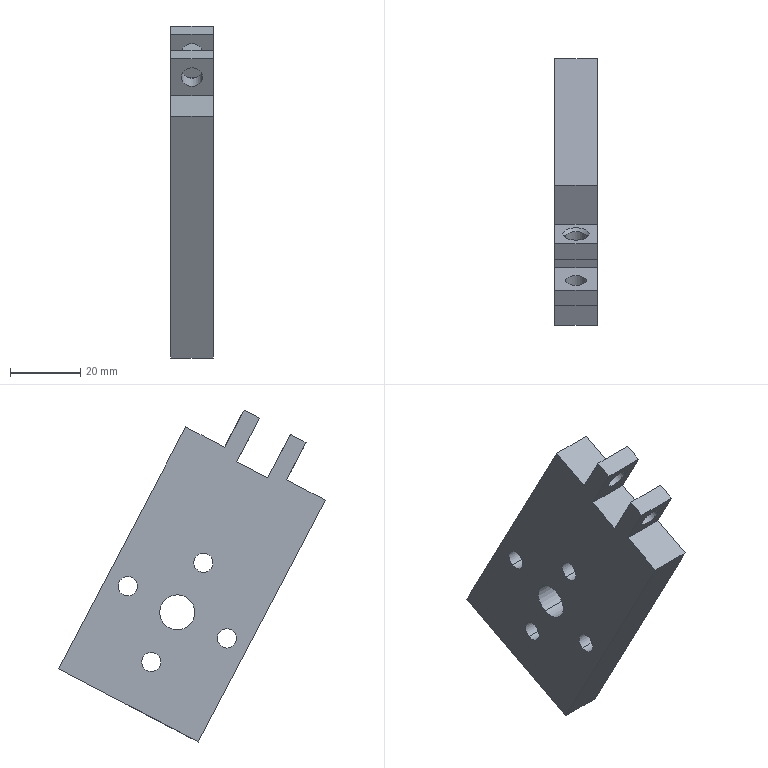Component | SolidWorks | RotaryCylinderFixingPlate-1 | 1 solid | 50 faces | box 12 x 76.1 x 94.79 mm | volume 39022 mm3 | cylinder 26 | plane 18 | cone 6 | commonest cylinder face diameters 10 x10 5.5 x8 4.2 x4 6 x4
build123d program:
from build123d import *

# Parameters (mm, degrees)
SKETCH1_W                                          = 90
SKETCH1_H                                          = 45
BOSS_EXTRUDE1_DEPTH                                = 12
HOLE_SIZE_ACCORDING_TO_TYPE_1_OF_HEXAG_D           = 5.5
HOLE_SIZE_ACCORDING_TO_TYPE_1_OF_HEXAG_CBORE_D     = 10
HOLE_SIZE_ACCORDING_TO_TYPE_1_OF_HEXAG_CBORE_DEPTH = 5.7
SKETCH5_R                                          = 5
CUT_EXTRUDE1_DEPTH                                 = 52.723
SKETCH6_W                                          = 12
SKETCH6_H                                          = 12.5
CUT_EXTRUDE2_DEPTH                                 = 52.723
SKETCH7_W                                          = 28
SKETCH7_H                                          = 10
CUT_EXTRUDE3_DEPTH                                 = 52.723
F_6_0_6_DIAMETER_HOLE1_D                           = 6
M5_TAPPED_HOLE1_D                                  = 4.2
M5_TAPPED_HOLE1_DEPTH                              = 24
M5_TAPPED_HOLE1_TIP                                = 1.262
CHAMFER1_SIZE                                      = 0.8


with BuildPart() as part:
    # Sketch1 → Boss-Extrude1 (new body)
    with BuildSketch(Plane.XY):
        Rectangle(SKETCH1_W, SKETCH1_H)
    extrude(amount=BOSS_EXTRUDE1_DEPTH)

    # Hole Size _according to_ Type 1 of Hexag (through all)
    with Locations(Plane.XY.offset(12)):
        with Locations((15, 16), (15, -16), (31, 0), (-1, 0)):
            CounterBoreHole(HOLE_SIZE_ACCORDING_TO_TYPE_1_OF_HEXAG_D / 2, HOLE_SIZE_ACCORDING_TO_TYPE_1_OF_HEXAG_CBORE_D / 2, HOLE_SIZE_ACCORDING_TO_TYPE_1_OF_HEXAG_CBORE_DEPTH)

    # Sketch5 → Cut-Extrude1 (cut, through all)
    with BuildSketch(Plane.XY.offset(12)):
        with Locations((15, 0)):
            Circle(SKETCH5_R)
    extrude(amount=-CUT_EXTRUDE1_DEPTH, mode=Mode.SUBTRACT)

    # Sketch6 → Cut-Extrude2 (cut, through all)
    with BuildSketch(Plane.XY.offset(12)):
        with Locations((-39, 16.25)):
            Rectangle(SKETCH6_W, SKETCH6_H)
        with Locations((-39, -16.25)):
            Rectangle(SKETCH6_W, SKETCH6_H)
    extrude(amount=-CUT_EXTRUDE2_DEPTH, mode=Mode.SUBTRACT)

    # Sketch7 → Cut-Extrude3 (cut, through all)
    with BuildSketch(Plane.XY.offset(12)):
        with Locations((-45, 0)):
            Rectangle(SKETCH7_W, SKETCH7_H)
    extrude(amount=-CUT_EXTRUDE3_DEPTH, mode=Mode.SUBTRACT)

    # 6.0 _6_ Diameter Hole1 (through all)
    with Locations(Plane(origin=(0, 10, 0), x_dir=(1, 0, 0), z_dir=(0, 1, 0))):
        with Locations((-39, -6)):
            Hole(F_6_0_6_DIAMETER_HOLE1_D / 2)

    # M5 Tapped Hole1
    with Locations(Plane(origin=(45, 0, 0), x_dir=(0, 0, -1), z_dir=(1, 0, 0))):
        with Locations((-6, 15), (-6, -15)):
            Hole(M5_TAPPED_HOLE1_D / 2, depth=M5_TAPPED_HOLE1_DEPTH)
            with Locations((0, 0, -(M5_TAPPED_HOLE1_DEPTH + M5_TAPPED_HOLE1_TIP / 2))):  # 118° drill point
                Cone(0, M5_TAPPED_HOLE1_D / 2, M5_TAPPED_HOLE1_TIP, mode=Mode.SUBTRACT)

    # Chamfer1
    chamfer1_edges = [part.edges().sort_by_distance(p)[0] for p in [
        (-36, 10, 6),
    ]]
    chamfer(chamfer1_edges, length=CHAMFER1_SIZE)


solid = part.part

# Placed as in the assembly
solid = solid.moved(Location((-279.317, -4.285, 137.993), (27.698, 90, 0)))